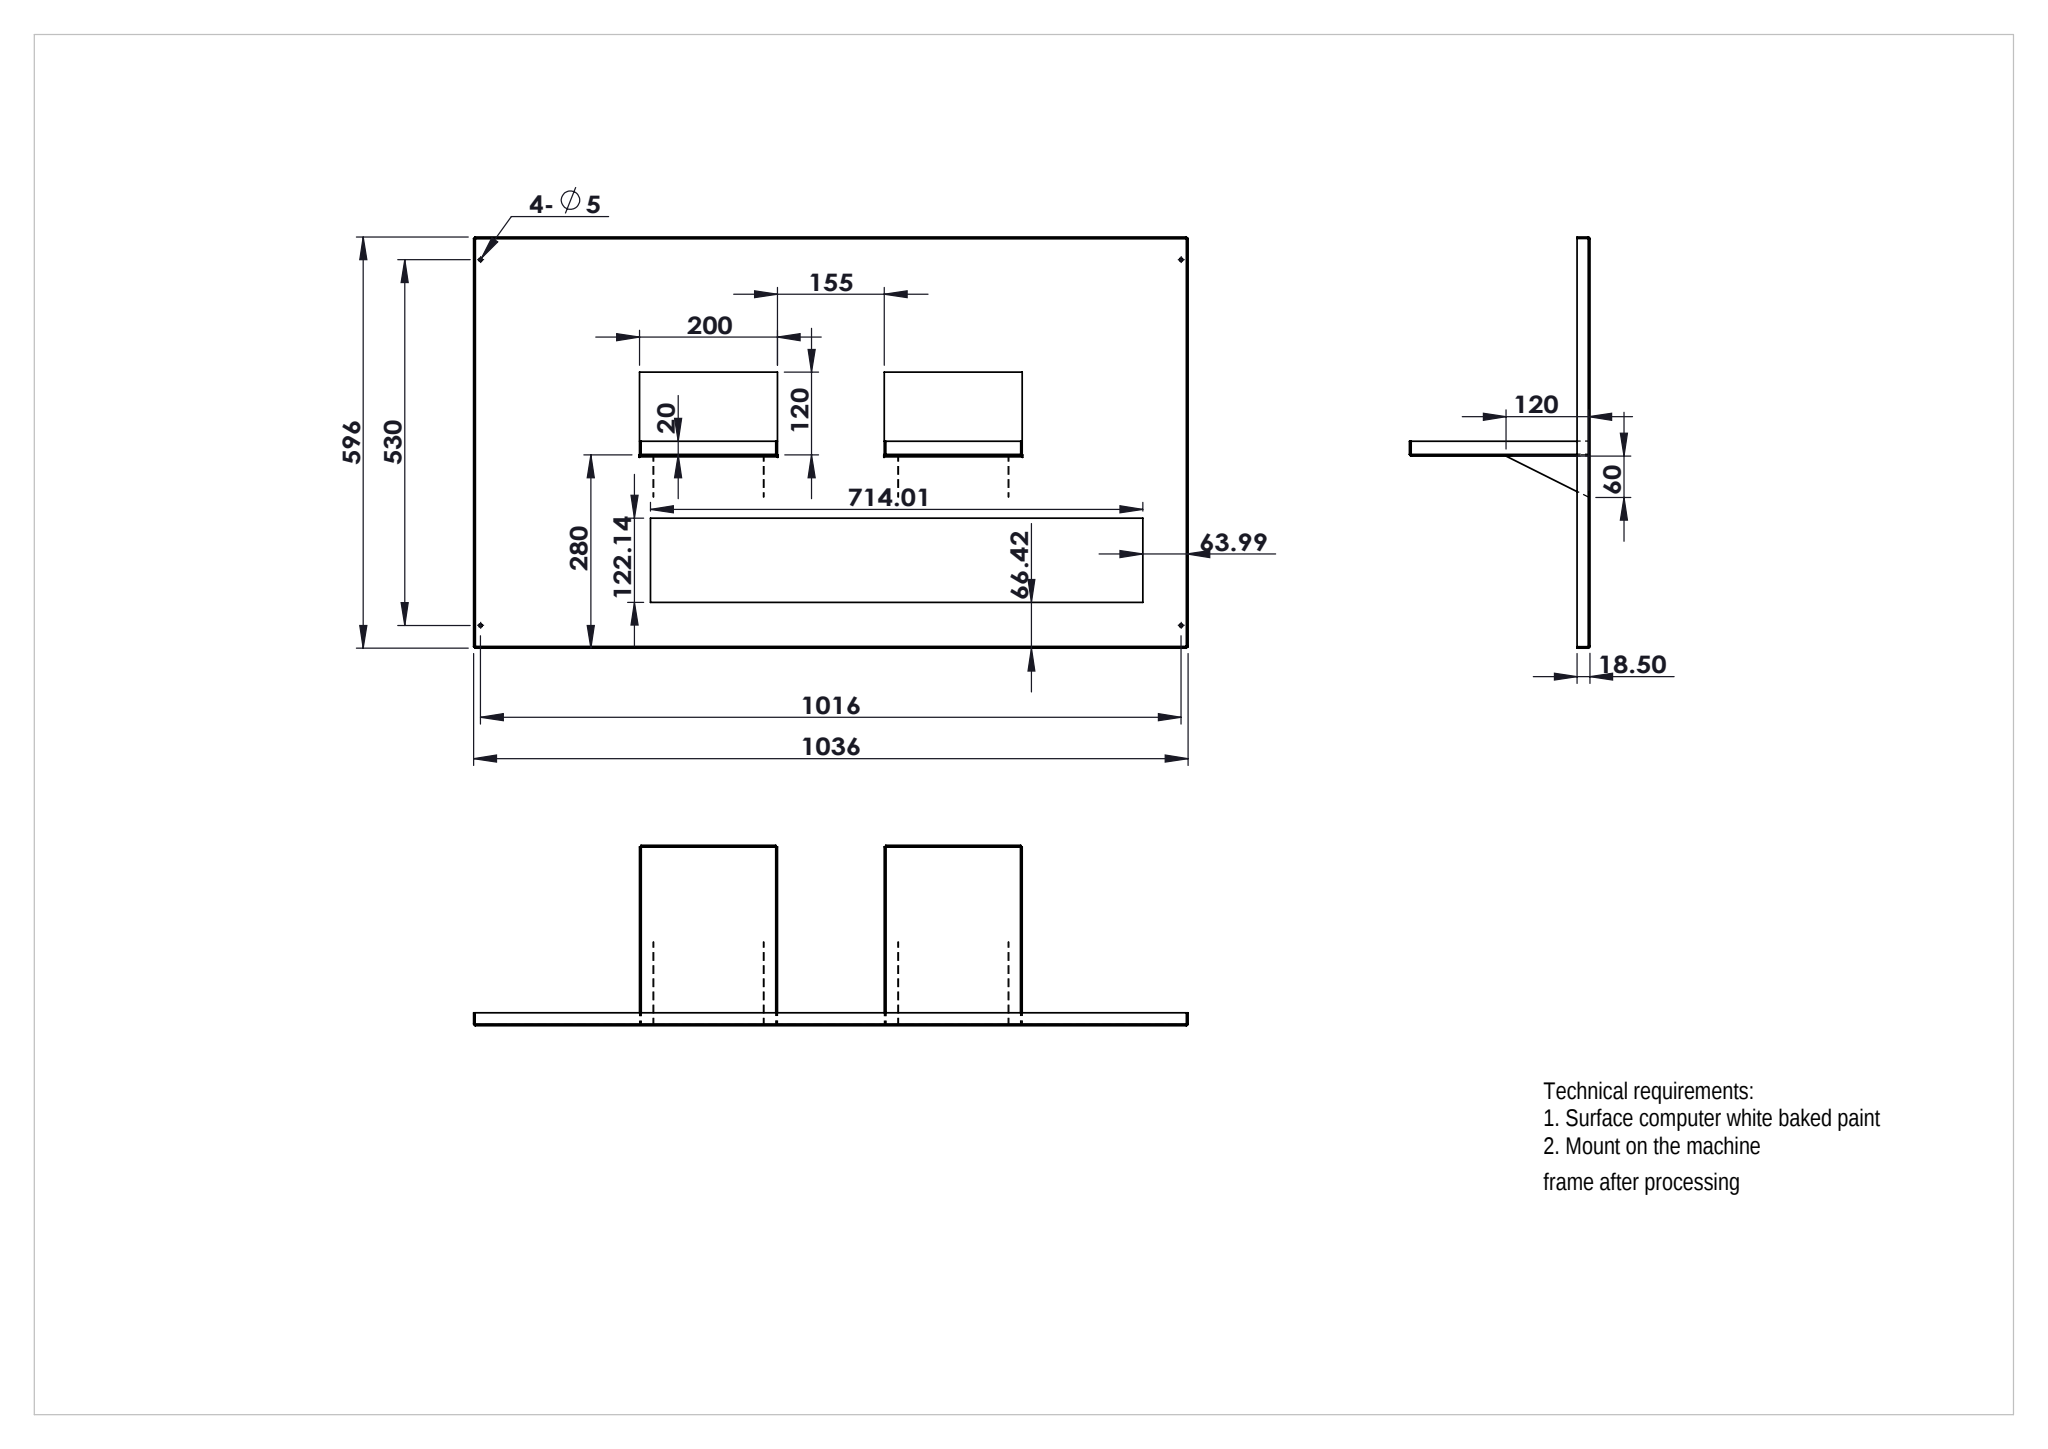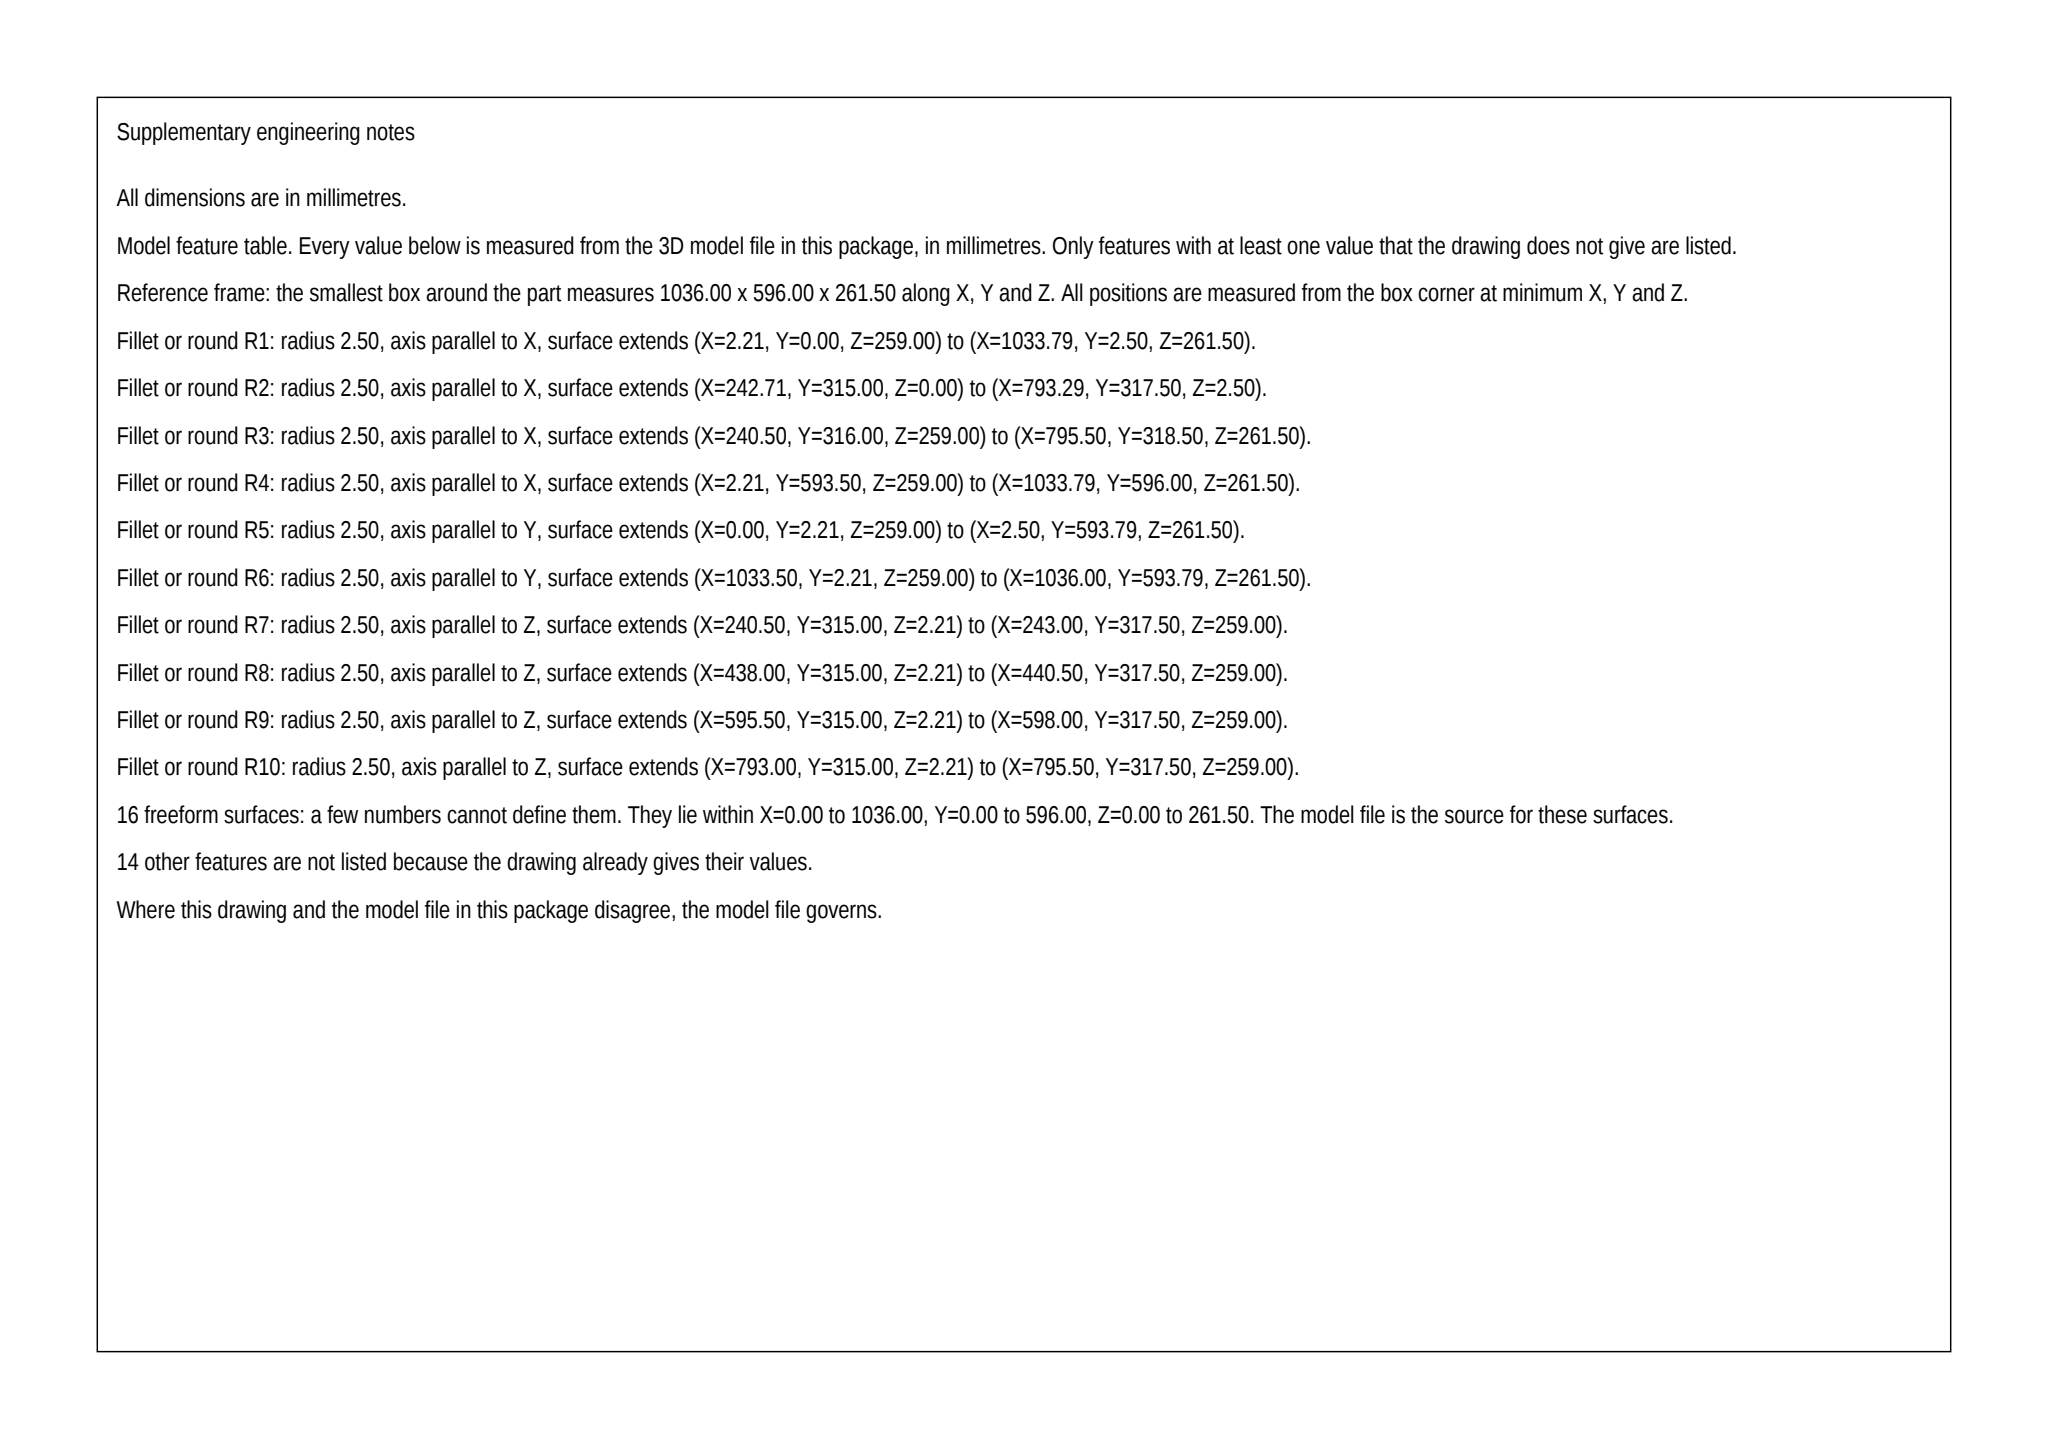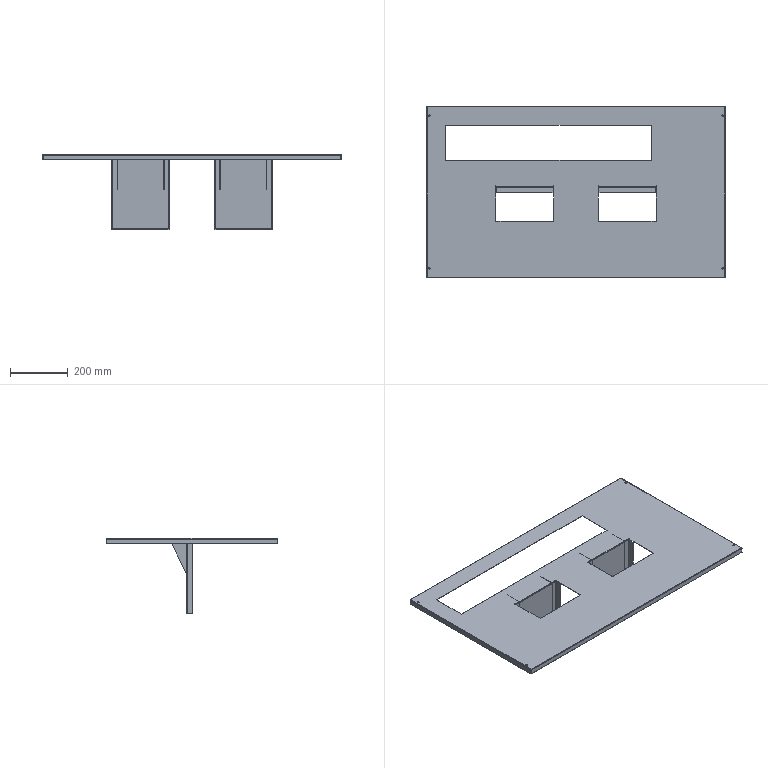Part | SolidWorks | mm | 1 solid | 158 faces | box 1036 x 596 x 261.5 mm | volume 1013191 mm3 | plane 106 | cylinder 36 | spline 16 | commonest cylinder face diameters 5 x20 2 x16
Drawing notes:
BRACKETS PROJECT 243 FROM PANEL REAR FACE; 261.5 OVERALL DEPTH | from the solid: Z planes: bracket base 0.02, panel rear face 243.02, front 261.52; bbox Z=261.53
BRACKET SHEET THK 1.5 | from the solid: Paired Z planes 0.02/1.52 and X planes 239.77-242.02, 1.5 wall offsets
240.5 FROM LH PANEL EDGE TO 1ST BRACKET; PAIR SYM ABOUT PANEL CL | from the solid: Bracket outer faces X=240.52 & 795.52 vs panel edges X=0.02 & 1036.02
ALL FRONT FACE PERIMETER EDGES R2.5 | from the solid: Ø5 edge cyls at y=2.52/593.52 & x=2.52/1033.52, z=259.02, len 1031.59/591.59
RECT CUTOUT 714.01 X 122.14 THRU 1.5 THK PANEL FACE | from the solid: Cutout walls x=65.51/779.52 (714.01), y=407.45/529.60 (122.15); panel face planes z=260.02 & 261.52 => 1.5 thk, no floor plane => thru
4X Ø5 THRU 1.5 THK PANEL FACE ( DP 1.5) | from the solid: Ø5 z-axis holes L=1.5 at (10.02,33.02),(10.02,563.02),(1026.02,33.02),(1026.02,563.02); face thickness z 260.02-261.52 = 1.5
BRACKETS PROJECT 260.0 FROM PANEL REAR FACE (BRACKET FREE END Z=0 TO PANEL REAR FACE Z=260.0); PART OVERALL DEPTH 261.5 | from the solid: z-planes 0.02 (bracket free end), 260.02 (panel rear face), 261.52 (panel front face); bbox_z 261.53
PANEL FACE PLATE 1.5 THK: FRONT FACE AT Z=261.5, REAR FACE AT Z=260.0 (SIDE-VIEW PLATE THICKNESS = 1.5, NOT 18.5) | from the solid: z-planes 260.02 and 261.52 (1.5 apart); notes agree with 1.5 THK panel face
2X INTERNAL WEB PER BRACKET, 1.0 THK, INNER FACES 19.5 FROM EACH BRACKET SIDE-WALL OUTER FACE, 159.0 CLEAR BETWEEN WEBS (160.0 CTR-CTR) | from the solid: x-planes 260.02/261.02 and 420.02/421.02 (bracket 1, outer faces 240.52/440.52); 615.02/616.02 and 775.02/776.02 (bracket 2, outer faces 595.52/795.52)
BRACKET SIDE WALLS 1.5 THK; EACH BRACKET 200.0 WIDE OVERALL, 1ST BRACKET AT X=240.5 FROM LH PANEL EDGE, 2ND AT X=595.5 (155.0 CLEAR BETWEEN BRACKETS) | from the solid: x-planes 240.52/242.02 and 439.02/440.52; 595.52/597.02 and 794.02/795.52
BRACKET END CLOSURE PLATE 1.5 THK AT BRACKET FREE END, Z=0 TO Z=1.5 (258.5 FROM PANEL REAR FACE) | from the solid: z-planes 0.02 and 1.52 (count 2 each) spanning bracket cross-section
INTERNAL STEP FACE IN EACH BRACKET AT Z=243.0, I.E. 17.0 FROM PANEL REAR FACE (Z=260.0) | from the solid: z-plane 243.02, count 4 (2 per bracket)
BRACKET VERTICAL CORNERS R2.5 OUTSIDE / R1 INSIDE AT X=243.0, 438.0, 598.0, 793.0; ALL OTHER UNSPECIFIED BRACKET EDGE BREAKS R1 | from the solid: z-axis cylinders dia 5.0 and dia 2.0 at (243.02,315.02),(438.02,315.02),(598.02,315.02),(793.02,315.02) L=256.79; dia 2.0 x-axis cylinders L=19.5/159.0 at y=318.52, z=259.02
RECTANGULAR CUTOUT CORNERS SHARP - NO CORNER RADIUS | from the solid: fillet_radii list empty and no cylinders at cutout corners (cutout x 65.51-779.52, y 407.45-529.60)
4X Ø5 THRU 1.5 THK PANEL FACE LOCATED 10.0 FROM LH AND RH PANEL EDGES AND 33.0 FROM TOP AND BOTTOM PANEL EDGES | from the solid: dia 5.0 z-axis cylinders L=1.5 at (10.02,33.02),(10.02,563.02),(1026.02,33.02),(1026.02,563.02) in 1036.03 x 596.03 panel